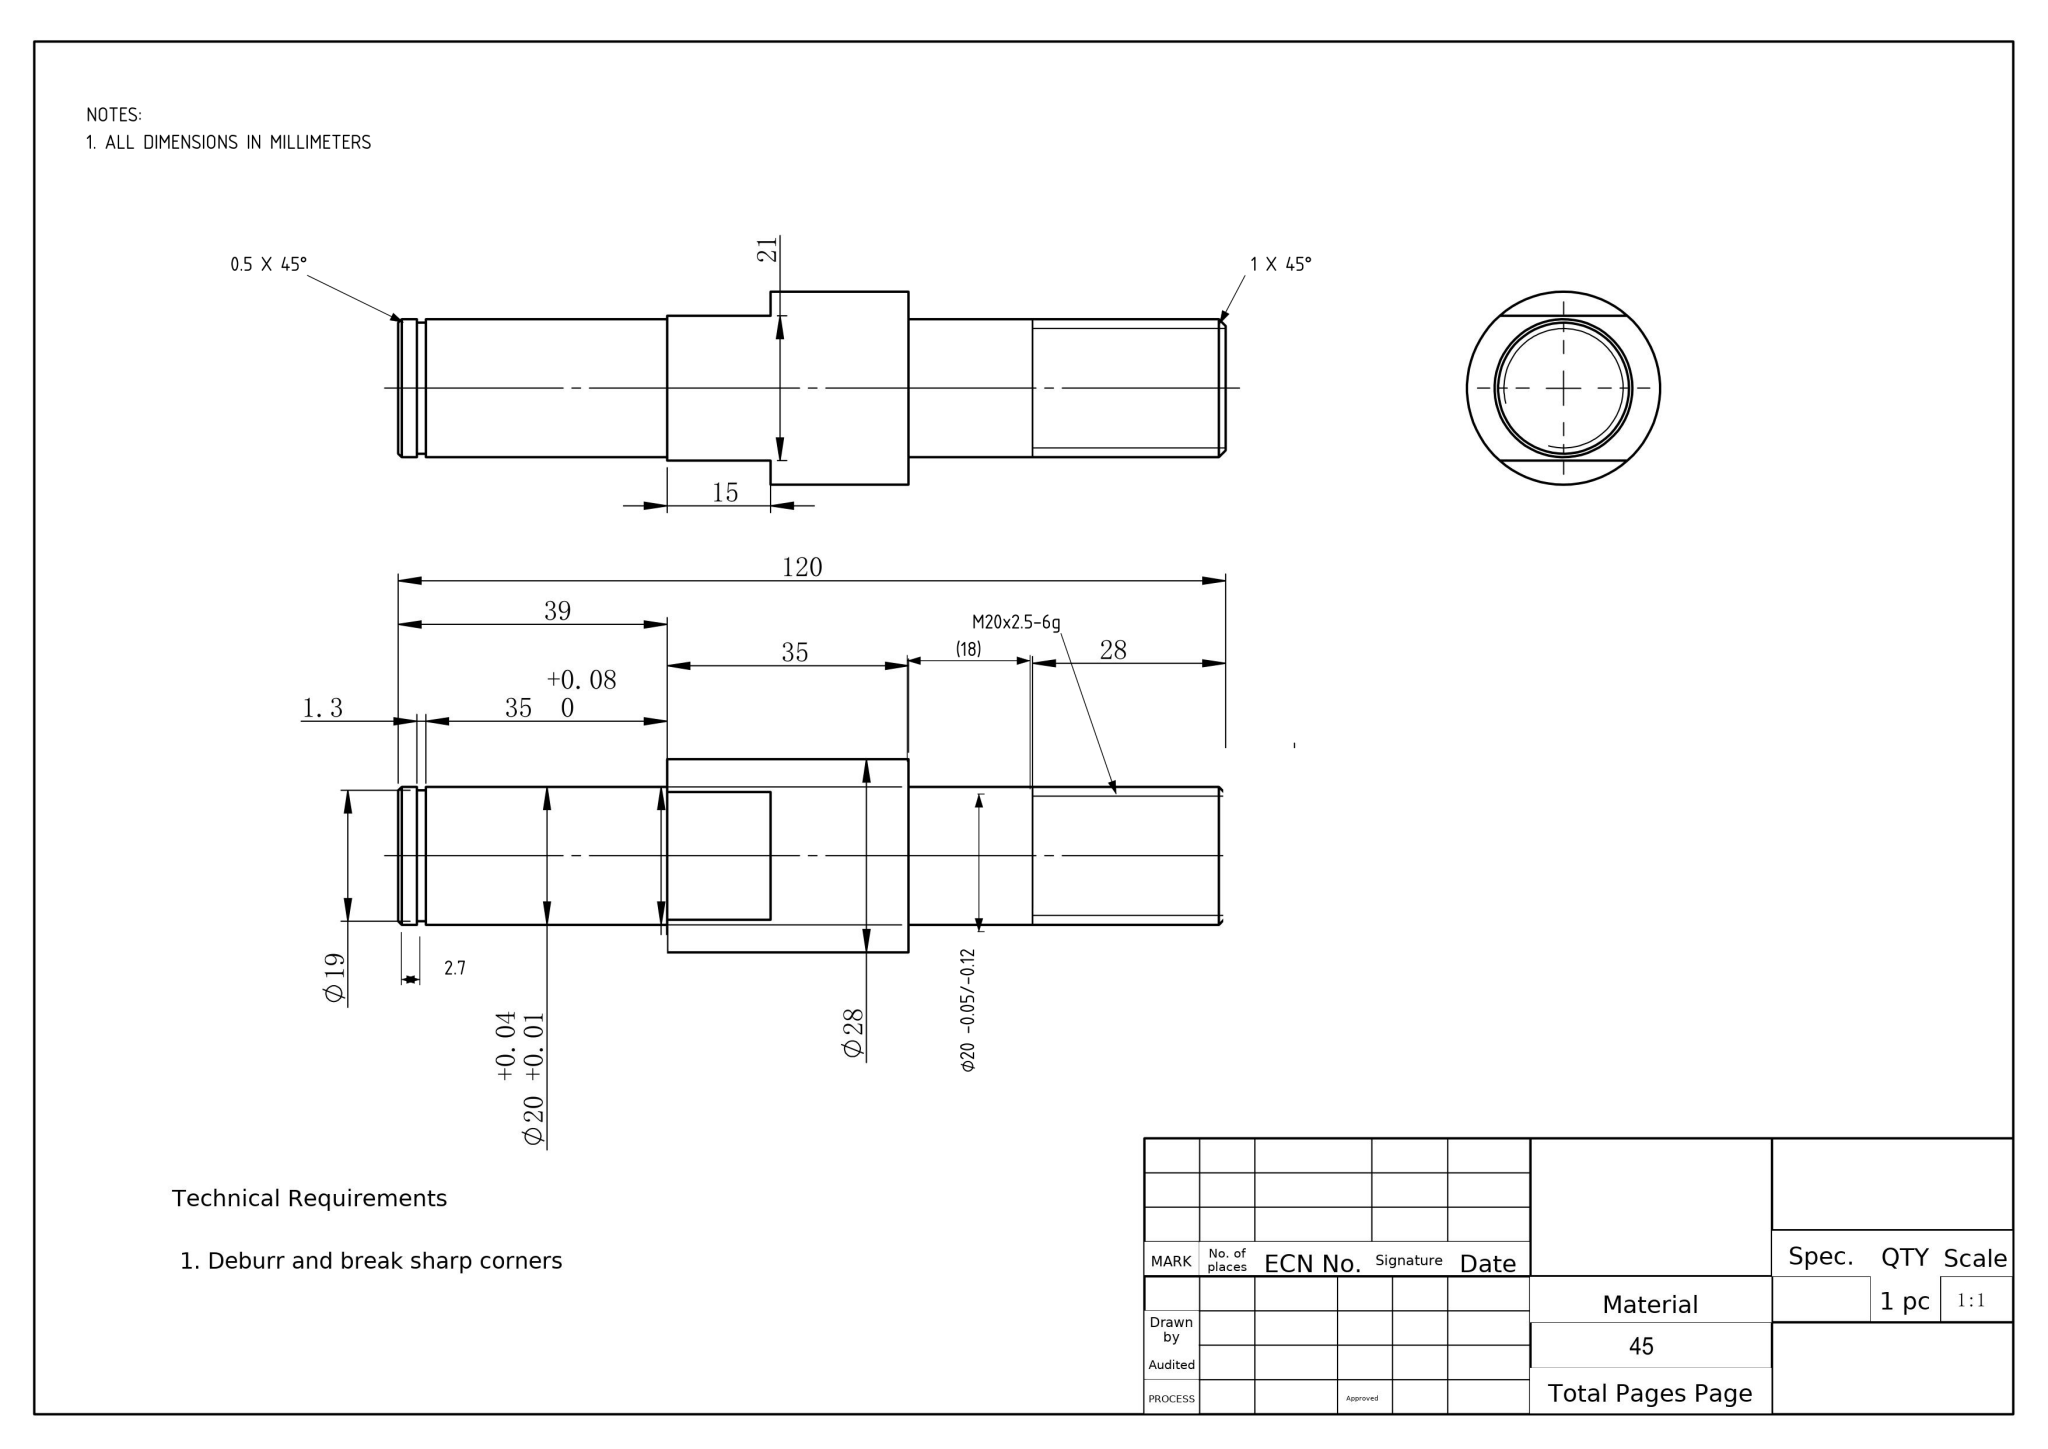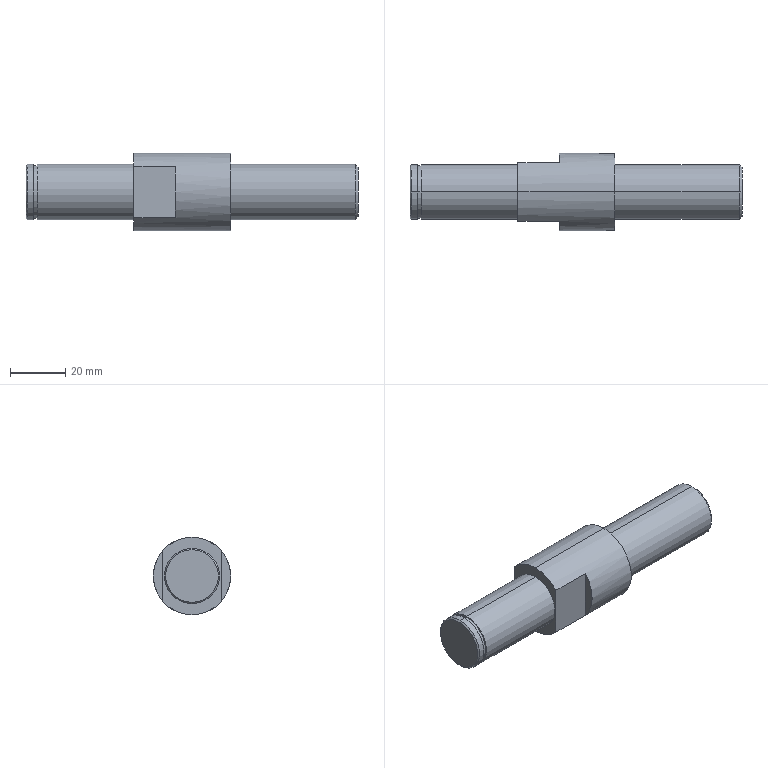Part | NX | mm | 1 solid | 24 faces | box 120 x 28 x 28 mm | volume 46844 mm3 | cylinder 10 | plane 10 | cone 4 | commonest cylinder face diameters 20 x6 19 x2 28 x2
STEP:
#1=COLOUR_RGB('',1.,0.502,0.502);
#2=FILL_AREA_STYLE_COLOUR('',#1);
#3=FILL_AREA_STYLE('',(#2));
#4=SURFACE_STYLE_FILL_AREA(#3);
#5=SURFACE_SIDE_STYLE('',(#4));
#6=SURFACE_STYLE_USAGE(.BOTH.,#5);
#7=PRESENTATION_STYLE_ASSIGNMENT((#6));
#8=CARTESIAN_POINT('',(120.,0.,9.));
#9=VERTEX_POINT('',#8);
#10=CARTESIAN_POINT('',(120.,0.,-9.));
#11=VERTEX_POINT('',#10);
#12=CARTESIAN_POINT('',(120.,0.,0.));
#13=DIRECTION('',(-1.,0.,0.));
#14=DIRECTION('',(0.,0.,1.));
#15=AXIS2_PLACEMENT_3D('',#12,#13,#14);
#16=CIRCLE('',#15,9.);
#17=EDGE_CURVE('',#9,#11,#16,.T.);
#18=ORIENTED_EDGE('',*,*,#17,.T.);
#19=CARTESIAN_POINT('',(119.,0.,-10.));
#20=VERTEX_POINT('',#19);
#21=CARTESIAN_POINT('',(120.,0.,-9.));
#22=DIRECTION('',(-0.7071,0.,-0.7071));
#23=VECTOR('',#22,1000.);
#24=LINE('',#21,#23);
#25=EDGE_CURVE('',#11,#20,#24,.T.);
#26=ORIENTED_EDGE('',*,*,#25,.T.);
#27=CARTESIAN_POINT('',(119.,0.,10.));
#28=VERTEX_POINT('',#27);
#29=CARTESIAN_POINT('',(119.,0.,0.));
#30=DIRECTION('',(-1.,0.,0.));
#31=DIRECTION('',(0.,0.,1.));
#32=AXIS2_PLACEMENT_3D('',#29,#30,#31);
#33=CIRCLE('',#32,10.);
#34=EDGE_CURVE('',#28,#20,#33,.T.);
#35=ORIENTED_EDGE('',*,*,#34,.F.);
#36=CARTESIAN_POINT('',(120.,0.,9.));
#37=DIRECTION('',(-0.7071,0.,0.7071));
#38=VECTOR('',#37,1000.);
#39=LINE('',#36,#38);
#40=EDGE_CURVE('',#9,#28,#39,.T.);
#41=ORIENTED_EDGE('',*,*,#40,.F.);
#42=EDGE_LOOP('',(#18,#26,#35,#41));
#43=FACE_OUTER_BOUND('',#42,.T.);
#44=CARTESIAN_POINT('',(120.,0.,0.));
#45=DIRECTION('',(-1.,0.,0.));
#46=DIRECTION('',(0.,0.,1.));
#47=AXIS2_PLACEMENT_3D('',#44,#45,#46);
#48=CONICAL_SURFACE('',#47,9.,0.7854);
#49=ADVANCED_FACE('',(#43),#48,.T.);
#50=ORIENTED_EDGE('',*,*,#34,.T.);
#51=CARTESIAN_POINT('',(74.,0.,-10.));
#52=VERTEX_POINT('',#51);
#53=CARTESIAN_POINT('',(0.,0.,-10.));
#54=DIRECTION('',(-1.,0.,0.));
#55=VECTOR('',#54,1000.);
#56=LINE('',#53,#55);
#57=EDGE_CURVE('',#20,#52,#56,.T.);
#58=ORIENTED_EDGE('',*,*,#57,.T.);
#59=CARTESIAN_POINT('',(74.,0.,10.));
#60=VERTEX_POINT('',#59);
#61=CARTESIAN_POINT('',(74.,0.,0.));
#62=DIRECTION('',(-1.,0.,0.));
#63=DIRECTION('',(0.,0.,1.));
#64=AXIS2_PLACEMENT_3D('',#61,#62,#63);
#65=CIRCLE('',#64,10.);
#66=EDGE_CURVE('',#60,#52,#65,.T.);
#67=ORIENTED_EDGE('',*,*,#66,.F.);
#68=CARTESIAN_POINT('',(0.,0.,10.));
#69=DIRECTION('',(-1.,0.,0.));
#70=VECTOR('',#69,1000.);
#71=LINE('',#68,#70);
#72=EDGE_CURVE('',#28,#60,#71,.T.);
#73=ORIENTED_EDGE('',*,*,#72,.F.);
#74=EDGE_LOOP('',(#50,#58,#67,#73));
#75=FACE_OUTER_BOUND('',#74,.T.);
#76=CARTESIAN_POINT('',(0.,0.,0.));
#77=DIRECTION('',(-1.,0.,0.));
#78=DIRECTION('',(0.,0.,1.));
#79=AXIS2_PLACEMENT_3D('',#76,#77,#78);
#80=CYLINDRICAL_SURFACE('',#79,10.);
#81=ADVANCED_FACE('',(#75),#80,.T.);
#82=CARTESIAN_POINT('',(39.,0.,10.));
#83=VERTEX_POINT('',#82);
#84=CARTESIAN_POINT('',(39.,0.,-10.));
#85=VERTEX_POINT('',#84);
#86=CARTESIAN_POINT('',(39.,0.,0.));
#87=DIRECTION('',(-1.,0.,0.));
#88=DIRECTION('',(0.,0.,1.));
#89=AXIS2_PLACEMENT_3D('',#86,#87,#88);
#90=CIRCLE('',#89,10.);
#91=EDGE_CURVE('',#83,#85,#90,.T.);
#92=ORIENTED_EDGE('',*,*,#91,.T.);
#93=CARTESIAN_POINT('',(4.,0.,-10.));
#94=VERTEX_POINT('',#93);
#95=CARTESIAN_POINT('',(0.,0.,-10.));
#96=DIRECTION('',(-1.,0.,0.));
#97=VECTOR('',#96,1000.);
#98=LINE('',#95,#97);
#99=EDGE_CURVE('',#85,#94,#98,.T.);
#100=ORIENTED_EDGE('',*,*,#99,.T.);
#101=CARTESIAN_POINT('',(4.,0.,10.));
#102=VERTEX_POINT('',#101);
#103=CARTESIAN_POINT('',(4.,0.,0.));
#104=DIRECTION('',(-1.,0.,0.));
#105=DIRECTION('',(0.,0.,1.));
#106=AXIS2_PLACEMENT_3D('',#103,#104,#105);
#107=CIRCLE('',#106,10.);
#108=EDGE_CURVE('',#102,#94,#107,.T.);
#109=ORIENTED_EDGE('',*,*,#108,.F.);
#110=CARTESIAN_POINT('',(0.,0.,10.));
#111=DIRECTION('',(-1.,0.,0.));
#112=VECTOR('',#111,1000.);
#113=LINE('',#110,#112);
#114=EDGE_CURVE('',#83,#102,#113,.T.);
#115=ORIENTED_EDGE('',*,*,#114,.F.);
#116=EDGE_LOOP('',(#92,#100,#109,#115));
#117=FACE_OUTER_BOUND('',#116,.T.);
#118=CARTESIAN_POINT('',(0.,0.,0.));
#119=DIRECTION('',(-1.,0.,0.));
#120=DIRECTION('',(0.,0.,1.));
#121=AXIS2_PLACEMENT_3D('',#118,#119,#120);
#122=CYLINDRICAL_SURFACE('',#121,10.);
#123=ADVANCED_FACE('',(#117),#122,.T.);
#124=CARTESIAN_POINT('',(4.,0.,9.5));
#125=VERTEX_POINT('',#124);
#126=CARTESIAN_POINT('',(4.,0.,-9.5));
#127=VERTEX_POINT('',#126);
#128=CARTESIAN_POINT('',(4.,0.,0.));
#129=DIRECTION('',(-1.,0.,0.));
#130=DIRECTION('',(0.,0.,1.));
#131=AXIS2_PLACEMENT_3D('',#128,#129,#130);
#132=CIRCLE('',#131,9.5);
#133=EDGE_CURVE('',#125,#127,#132,.T.);
#134=ORIENTED_EDGE('',*,*,#133,.T.);
#135=CARTESIAN_POINT('',(2.7,0.,-9.5));
#136=VERTEX_POINT('',#135);
#137=CARTESIAN_POINT('',(0.,0.,-9.5));
#138=DIRECTION('',(-1.,0.,0.));
#139=VECTOR('',#138,1000.);
#140=LINE('',#137,#139);
#141=EDGE_CURVE('',#127,#136,#140,.T.);
#142=ORIENTED_EDGE('',*,*,#141,.T.);
#143=CARTESIAN_POINT('',(2.7,0.,9.5));
#144=VERTEX_POINT('',#143);
#145=CARTESIAN_POINT('',(2.7,0.,0.));
#146=DIRECTION('',(-1.,0.,0.));
#147=DIRECTION('',(0.,0.,1.));
#148=AXIS2_PLACEMENT_3D('',#145,#146,#147);
#149=CIRCLE('',#148,9.5);
#150=EDGE_CURVE('',#144,#136,#149,.T.);
#151=ORIENTED_EDGE('',*,*,#150,.F.);
#152=CARTESIAN_POINT('',(0.,0.,9.5));
#153=DIRECTION('',(-1.,0.,0.));
#154=VECTOR('',#153,1000.);
#155=LINE('',#152,#154);
#156=EDGE_CURVE('',#125,#144,#155,.T.);
#157=ORIENTED_EDGE('',*,*,#156,.F.);
#158=EDGE_LOOP('',(#134,#142,#151,#157));
#159=FACE_OUTER_BOUND('',#158,.T.);
#160=CARTESIAN_POINT('',(0.,0.,0.));
#161=DIRECTION('',(-1.,0.,0.));
#162=DIRECTION('',(0.,0.,1.));
#163=AXIS2_PLACEMENT_3D('',#160,#161,#162);
#164=CYLINDRICAL_SURFACE('',#163,9.5);
#165=ADVANCED_FACE('',(#159),#164,.T.);
#166=CARTESIAN_POINT('',(2.7,0.,10.));
#167=VERTEX_POINT('',#166);
#168=CARTESIAN_POINT('',(2.7,0.,-10.));
#169=VERTEX_POINT('',#168);
#170=CARTESIAN_POINT('',(2.7,0.,0.));
#171=DIRECTION('',(-1.,0.,0.));
#172=DIRECTION('',(0.,0.,1.));
#173=AXIS2_PLACEMENT_3D('',#170,#171,#172);
#174=CIRCLE('',#173,10.);
#175=EDGE_CURVE('',#167,#169,#174,.T.);
#176=ORIENTED_EDGE('',*,*,#175,.T.);
#177=CARTESIAN_POINT('',(0.5,0.,-10.));
#178=VERTEX_POINT('',#177);
#179=CARTESIAN_POINT('',(0.,0.,-10.));
#180=DIRECTION('',(-1.,0.,0.));
#181=VECTOR('',#180,1000.);
#182=LINE('',#179,#181);
#183=EDGE_CURVE('',#169,#178,#182,.T.);
#184=ORIENTED_EDGE('',*,*,#183,.T.);
#185=CARTESIAN_POINT('',(0.5,0.,10.));
#186=VERTEX_POINT('',#185);
#187=CARTESIAN_POINT('',(0.5,0.,0.));
#188=DIRECTION('',(-1.,0.,0.));
#189=DIRECTION('',(0.,0.,1.));
#190=AXIS2_PLACEMENT_3D('',#187,#188,#189);
#191=CIRCLE('',#190,10.);
#192=EDGE_CURVE('',#186,#178,#191,.T.);
#193=ORIENTED_EDGE('',*,*,#192,.F.);
#194=CARTESIAN_POINT('',(0.,0.,10.));
#195=DIRECTION('',(-1.,0.,0.));
#196=VECTOR('',#195,1000.);
#197=LINE('',#194,#196);
#198=EDGE_CURVE('',#167,#186,#197,.T.);
#199=ORIENTED_EDGE('',*,*,#198,.F.);
#200=EDGE_LOOP('',(#176,#184,#193,#199));
#201=FACE_OUTER_BOUND('',#200,.T.);
#202=CARTESIAN_POINT('',(0.,0.,0.));
#203=DIRECTION('',(-1.,0.,0.));
#204=DIRECTION('',(0.,0.,1.));
#205=AXIS2_PLACEMENT_3D('',#202,#203,#204);
#206=CYLINDRICAL_SURFACE('',#205,10.);
#207=ADVANCED_FACE('',(#201),#206,.T.);
#208=CARTESIAN_POINT('',(0.,0.,9.5));
#209=VERTEX_POINT('',#208);
#210=CARTESIAN_POINT('',(0.,0.,-9.5));
#211=VERTEX_POINT('',#210);
#212=CARTESIAN_POINT('',(0.,0.,0.));
#213=DIRECTION('',(-1.,0.,0.));
#214=DIRECTION('',(0.,0.,1.));
#215=AXIS2_PLACEMENT_3D('',#212,#213,#214);
#216=CIRCLE('',#215,9.5);
#217=EDGE_CURVE('',#209,#211,#216,.T.);
#218=ORIENTED_EDGE('',*,*,#217,.F.);
#219=CARTESIAN_POINT('',(0.5,0.,10.));
#220=DIRECTION('',(0.7071,0.,0.7071));
#221=VECTOR('',#220,1000.);
#222=LINE('',#219,#221);
#223=EDGE_CURVE('',#209,#186,#222,.T.);
#224=ORIENTED_EDGE('',*,*,#223,.T.);
#225=ORIENTED_EDGE('',*,*,#192,.T.);
#226=CARTESIAN_POINT('',(0.5,0.,-10.));
#227=DIRECTION('',(0.7071,0.,-0.7071));
#228=VECTOR('',#227,1000.);
#229=LINE('',#226,#228);
#230=EDGE_CURVE('',#211,#178,#229,.T.);
#231=ORIENTED_EDGE('',*,*,#230,.F.);
#232=EDGE_LOOP('',(#218,#224,#225,#231));
#233=FACE_OUTER_BOUND('',#232,.T.);
#234=CARTESIAN_POINT('',(0.5,0.,0.));
#235=DIRECTION('',(1.,0.,0.));
#236=DIRECTION('',(0.,0.,-1.));
#237=AXIS2_PLACEMENT_3D('',#234,#235,#236);
#238=CONICAL_SURFACE('',#237,10.,0.7854);
#239=ADVANCED_FACE('',(#233),#238,.T.);
#240=CARTESIAN_POINT('',(74.,0.,14.));
#241=VERTEX_POINT('',#240);
#242=CARTESIAN_POINT('',(74.,0.,-14.));
#243=VERTEX_POINT('',#242);
#244=CARTESIAN_POINT('',(74.,0.,0.));
#245=DIRECTION('',(-1.,0.,0.));
#246=DIRECTION('',(0.,0.,1.));
#247=AXIS2_PLACEMENT_3D('',#244,#245,#246);
#248=CIRCLE('',#247,14.);
#249=EDGE_CURVE('',#241,#243,#248,.T.);
#250=ORIENTED_EDGE('',*,*,#249,.T.);
#251=CARTESIAN_POINT('',(39.,0.,-14.));
#252=VERTEX_POINT('',#251);
#253=CARTESIAN_POINT('',(0.,0.,-14.));
#254=DIRECTION('',(-1.,0.,0.));
#255=VECTOR('',#254,1000.);
#256=LINE('',#253,#255);
#257=EDGE_CURVE('',#243,#252,#256,.T.);
#258=ORIENTED_EDGE('',*,*,#257,.T.);
#259=CARTESIAN_POINT('',(39.,10.5,-9.26));
#260=VERTEX_POINT('',#259);
#261=CARTESIAN_POINT('',(39.,0.,0.));
#262=DIRECTION('',(-1.,0.,0.));
#263=DIRECTION('',(0.,0.,1.));
#264=AXIS2_PLACEMENT_3D('',#261,#262,#263);
#265=CIRCLE('',#264,14.);
#266=EDGE_CURVE('',#260,#252,#265,.T.);
#267=ORIENTED_EDGE('',*,*,#266,.F.);
#268=CARTESIAN_POINT('',(54.,10.5,-9.26));
#269=VERTEX_POINT('',#268);
#270=CARTESIAN_POINT('',(0.,10.5,-9.26));
#271=DIRECTION('',(-1.,0.,0.));
#272=VECTOR('',#271,1000.);
#273=LINE('',#270,#272);
#274=EDGE_CURVE('',#269,#260,#273,.T.);
#275=ORIENTED_EDGE('',*,*,#274,.F.);
#276=CARTESIAN_POINT('',(54.,10.5,9.26));
#277=VERTEX_POINT('',#276);
#278=CARTESIAN_POINT('',(54.,0.,0.));
#279=DIRECTION('',(-1.,0.,0.));
#280=DIRECTION('',(0.,0.,1.));
#281=AXIS2_PLACEMENT_3D('',#278,#279,#280);
#282=CIRCLE('',#281,14.);
#283=EDGE_CURVE('',#277,#269,#282,.T.);
#284=ORIENTED_EDGE('',*,*,#283,.F.);
#285=CARTESIAN_POINT('',(39.,10.5,9.26));
#286=VERTEX_POINT('',#285);
#287=CARTESIAN_POINT('',(0.,10.5,9.26));
#288=DIRECTION('',(1.,0.,0.));
#289=VECTOR('',#288,1000.);
#290=LINE('',#287,#289);
#291=EDGE_CURVE('',#286,#277,#290,.T.);
#292=ORIENTED_EDGE('',*,*,#291,.F.);
#293=CARTESIAN_POINT('',(39.,0.,14.));
#294=VERTEX_POINT('',#293);
#295=CARTESIAN_POINT('',(39.,0.,0.));
#296=DIRECTION('',(-1.,0.,0.));
#297=DIRECTION('',(0.,0.,1.));
#298=AXIS2_PLACEMENT_3D('',#295,#296,#297);
#299=CIRCLE('',#298,14.);
#300=EDGE_CURVE('',#294,#286,#299,.T.);
#301=ORIENTED_EDGE('',*,*,#300,.F.);
#302=CARTESIAN_POINT('',(0.,0.,14.));
#303=DIRECTION('',(-1.,0.,0.));
#304=VECTOR('',#303,1000.);
#305=LINE('',#302,#304);
#306=EDGE_CURVE('',#241,#294,#305,.T.);
#307=ORIENTED_EDGE('',*,*,#306,.F.);
#308=EDGE_LOOP('',(#250,#258,#267,#275,#284,#292,#301,#307));
#309=FACE_OUTER_BOUND('',#308,.T.);
#310=CARTESIAN_POINT('',(0.,0.,0.));
#311=DIRECTION('',(-1.,0.,0.));
#312=DIRECTION('',(0.,0.,1.));
#313=AXIS2_PLACEMENT_3D('',#310,#311,#312);
#314=CYLINDRICAL_SURFACE('',#313,14.);
#315=ADVANCED_FACE('',(#309),#314,.T.);
#316=ORIENTED_EDGE('',*,*,#91,.F.);
#317=CARTESIAN_POINT('',(39.,0.,0.));
#318=DIRECTION('',(-1.,0.,0.));
#319=DIRECTION('',(0.,0.,1.));
#320=AXIS2_PLACEMENT_3D('',#317,#318,#319);
#321=CIRCLE('',#320,10.);
#322=EDGE_CURVE('',#85,#83,#321,.T.);
#323=ORIENTED_EDGE('',*,*,#322,.F.);
#324=EDGE_LOOP('',(#316,#323));
#325=FACE_BOUND('',#324,.T.);
#326=CARTESIAN_POINT('',(39.,-10.5,-9.26));
#327=VERTEX_POINT('',#326);
#328=CARTESIAN_POINT('',(39.,-10.5,9.26));
#329=VERTEX_POINT('',#328);
#330=CARTESIAN_POINT('',(39.,-10.5,-15.599));
#331=DIRECTION('',(0.,0.,1.));
#332=VECTOR('',#331,1000.);
#333=LINE('',#330,#332);
#334=EDGE_CURVE('',#327,#329,#333,.T.);
#335=ORIENTED_EDGE('',*,*,#334,.T.);
#336=CARTESIAN_POINT('',(39.,0.,0.));
#337=DIRECTION('',(-1.,0.,0.));
#338=DIRECTION('',(0.,0.,1.));
#339=AXIS2_PLACEMENT_3D('',#336,#337,#338);
#340=CIRCLE('',#339,14.);
#341=EDGE_CURVE('',#329,#294,#340,.T.);
#342=ORIENTED_EDGE('',*,*,#341,.T.);
#343=ORIENTED_EDGE('',*,*,#300,.T.);
#344=CARTESIAN_POINT('',(39.,10.5,-15.599));
#345=DIRECTION('',(0.,0.,-1.));
#346=VECTOR('',#345,1000.);
#347=LINE('',#344,#346);
#348=EDGE_CURVE('',#286,#260,#347,.T.);
#349=ORIENTED_EDGE('',*,*,#348,.T.);
#350=ORIENTED_EDGE('',*,*,#266,.T.);
#351=CARTESIAN_POINT('',(39.,0.,0.));
#352=DIRECTION('',(-1.,0.,0.));
#353=DIRECTION('',(0.,0.,1.));
#354=AXIS2_PLACEMENT_3D('',#351,#352,#353);
#355=CIRCLE('',#354,14.);
#356=EDGE_CURVE('',#252,#327,#355,.T.);
#357=ORIENTED_EDGE('',*,*,#356,.T.);
#358=EDGE_LOOP('',(#335,#342,#343,#349,#350,#357));
#359=FACE_OUTER_BOUND('',#358,.T.);
#360=CARTESIAN_POINT('',(39.,10.,0.));
#361=DIRECTION('',(1.,0.,0.));
#362=DIRECTION('',(0.,0.,-1.));
#363=AXIS2_PLACEMENT_3D('',#360,#361,#362);
#364=PLANE('',#363);
#365=ADVANCED_FACE('',(#325,#359),#364,.F.);
#366=ORIENTED_EDGE('',*,*,#257,.F.);
#367=CARTESIAN_POINT('',(74.,0.,0.));
#368=DIRECTION('',(-1.,0.,0.));
#369=DIRECTION('',(0.,0.,1.));
#370=AXIS2_PLACEMENT_3D('',#367,#368,#369);
#371=CIRCLE('',#370,14.);
#372=EDGE_CURVE('',#243,#241,#371,.T.);
#373=ORIENTED_EDGE('',*,*,#372,.T.);
#374=ORIENTED_EDGE('',*,*,#306,.T.);
#375=ORIENTED_EDGE('',*,*,#341,.F.);
#376=CARTESIAN_POINT('',(54.,-10.5,9.26));
#377=VERTEX_POINT('',#376);
#378=CARTESIAN_POINT('',(0.,-10.5,9.26));
#379=DIRECTION('',(-1.,0.,0.));
#380=VECTOR('',#379,1000.);
#381=LINE('',#378,#380);
#382=EDGE_CURVE('',#377,#329,#381,.T.);
#383=ORIENTED_EDGE('',*,*,#382,.F.);
#384=CARTESIAN_POINT('',(54.,-10.5,-9.26));
#385=VERTEX_POINT('',#384);
#386=CARTESIAN_POINT('',(54.,0.,0.));
#387=DIRECTION('',(-1.,0.,0.));
#388=DIRECTION('',(0.,0.,1.));
#389=AXIS2_PLACEMENT_3D('',#386,#387,#388);
#390=CIRCLE('',#389,14.);
#391=EDGE_CURVE('',#385,#377,#390,.T.);
#392=ORIENTED_EDGE('',*,*,#391,.F.);
#393=CARTESIAN_POINT('',(0.,-10.5,-9.26));
#394=DIRECTION('',(1.,0.,0.));
#395=VECTOR('',#394,1000.);
#396=LINE('',#393,#395);
#397=EDGE_CURVE('',#327,#385,#396,.T.);
#398=ORIENTED_EDGE('',*,*,#397,.F.);
#399=ORIENTED_EDGE('',*,*,#356,.F.);
#400=EDGE_LOOP('',(#366,#373,#374,#375,#383,#392,#398,#399));
#401=FACE_OUTER_BOUND('',#400,.T.);
#402=CARTESIAN_POINT('',(0.,0.,0.));
#403=DIRECTION('',(-1.,0.,0.));
#404=DIRECTION('',(0.,0.,1.));
#405=AXIS2_PLACEMENT_3D('',#402,#403,#404);
#406=CYLINDRICAL_SURFACE('',#405,14.);
#407=ADVANCED_FACE('',(#401),#406,.T.);
#408=CARTESIAN_POINT('',(0.,0.,0.));
#409=DIRECTION('',(-1.,0.,0.));
#410=DIRECTION('',(0.,0.,1.));
#411=AXIS2_PLACEMENT_3D('',#408,#409,#410);
#412=CIRCLE('',#411,9.5);
#413=EDGE_CURVE('',#211,#209,#412,.T.);
#414=ORIENTED_EDGE('',*,*,#413,.T.);
#415=ORIENTED_EDGE('',*,*,#217,.T.);
#416=EDGE_LOOP('',(#414,#415));
#417=FACE_OUTER_BOUND('',#416,.T.);
#418=CARTESIAN_POINT('',(0.,0.,0.));
#419=DIRECTION('',(1.,0.,0.));
#420=DIRECTION('',(0.,0.,-1.));
#421=AXIS2_PLACEMENT_3D('',#418,#419,#420);
#422=PLANE('',#421);
#423=ADVANCED_FACE('',(#417),#422,.F.);
#424=ORIENTED_EDGE('',*,*,#223,.F.);
#425=ORIENTED_EDGE('',*,*,#413,.F.);
#426=ORIENTED_EDGE('',*,*,#230,.T.);
#427=CARTESIAN_POINT('',(0.5,0.,0.));
#428=DIRECTION('',(-1.,0.,0.));
#429=DIRECTION('',(0.,0.,1.));
#430=AXIS2_PLACEMENT_3D('',#427,#428,#429);
#431=CIRCLE('',#430,10.);
#432=EDGE_CURVE('',#178,#186,#431,.T.);
#433=ORIENTED_EDGE('',*,*,#432,.T.);
#434=EDGE_LOOP('',(#424,#425,#426,#433));
#435=FACE_OUTER_BOUND('',#434,.T.);
#436=CARTESIAN_POINT('',(0.5,0.,0.));
#437=DIRECTION('',(1.,0.,0.));
#438=DIRECTION('',(0.,0.,-1.));
#439=AXIS2_PLACEMENT_3D('',#436,#437,#438);
#440=CONICAL_SURFACE('',#439,10.,0.7854);
#441=ADVANCED_FACE('',(#435),#440,.T.);
#442=ORIENTED_EDGE('',*,*,#183,.F.);
#443=CARTESIAN_POINT('',(2.7,0.,0.));
#444=DIRECTION('',(-1.,0.,0.));
#445=DIRECTION('',(0.,0.,1.));
#446=AXIS2_PLACEMENT_3D('',#443,#444,#445);
#447=CIRCLE('',#446,10.);
#448=EDGE_CURVE('',#169,#167,#447,.T.);
#449=ORIENTED_EDGE('',*,*,#448,.T.);
#450=ORIENTED_EDGE('',*,*,#198,.T.);
#451=ORIENTED_EDGE('',*,*,#432,.F.);
#452=EDGE_LOOP('',(#442,#449,#450,#451));
#453=FACE_OUTER_BOUND('',#452,.T.);
#454=CARTESIAN_POINT('',(0.,0.,0.));
#455=DIRECTION('',(-1.,0.,0.));
#456=DIRECTION('',(0.,0.,1.));
#457=AXIS2_PLACEMENT_3D('',#454,#455,#456);
#458=CYLINDRICAL_SURFACE('',#457,10.);
#459=ADVANCED_FACE('',(#453),#458,.T.);
#460=ORIENTED_EDGE('',*,*,#175,.F.);
#461=ORIENTED_EDGE('',*,*,#448,.F.);
#462=EDGE_LOOP('',(#460,#461));
#463=FACE_OUTER_BOUND('',#462,.T.);
#464=ORIENTED_EDGE('',*,*,#150,.T.);
#465=CARTESIAN_POINT('',(2.7,0.,0.));
#466=DIRECTION('',(-1.,0.,0.));
#467=DIRECTION('',(0.,0.,1.));
#468=AXIS2_PLACEMENT_3D('',#465,#466,#467);
#469=CIRCLE('',#468,9.5);
#470=EDGE_CURVE('',#136,#144,#469,.T.);
#471=ORIENTED_EDGE('',*,*,#470,.T.);
#472=EDGE_LOOP('',(#464,#471));
#473=FACE_BOUND('',#472,.T.);
#474=CARTESIAN_POINT('',(2.7,10.,0.));
#475=DIRECTION('',(-1.,0.,0.));
#476=DIRECTION('',(0.,0.,1.));
#477=AXIS2_PLACEMENT_3D('',#474,#475,#476);
#478=PLANE('',#477);
#479=ADVANCED_FACE('',(#463,#473),#478,.F.);
#480=ORIENTED_EDGE('',*,*,#141,.F.);
#481=CARTESIAN_POINT('',(4.,0.,0.));
#482=DIRECTION('',(-1.,0.,0.));
#483=DIRECTION('',(0.,0.,1.));
#484=AXIS2_PLACEMENT_3D('',#481,#482,#483);
#485=CIRCLE('',#484,9.5);
#486=EDGE_CURVE('',#127,#125,#485,.T.);
#487=ORIENTED_EDGE('',*,*,#486,.T.);
#488=ORIENTED_EDGE('',*,*,#156,.T.);
#489=ORIENTED_EDGE('',*,*,#470,.F.);
#490=EDGE_LOOP('',(#480,#487,#488,#489));
#491=FACE_OUTER_BOUND('',#490,.T.);
#492=CARTESIAN_POINT('',(0.,0.,0.));
#493=DIRECTION('',(-1.,0.,0.));
#494=DIRECTION('',(0.,0.,1.));
#495=AXIS2_PLACEMENT_3D('',#492,#493,#494);
#496=CYLINDRICAL_SURFACE('',#495,9.5);
#497=ADVANCED_FACE('',(#491),#496,.T.);
#498=ORIENTED_EDGE('',*,*,#133,.F.);
#499=ORIENTED_EDGE('',*,*,#486,.F.);
#500=EDGE_LOOP('',(#498,#499));
#501=FACE_BOUND('',#500,.T.);
#502=ORIENTED_EDGE('',*,*,#108,.T.);
#503=CARTESIAN_POINT('',(4.,0.,0.));
#504=DIRECTION('',(-1.,0.,0.));
#505=DIRECTION('',(0.,0.,1.));
#506=AXIS2_PLACEMENT_3D('',#503,#504,#505);
#507=CIRCLE('',#506,10.);
#508=EDGE_CURVE('',#94,#102,#507,.T.);
#509=ORIENTED_EDGE('',*,*,#508,.T.);
#510=EDGE_LOOP('',(#502,#509));
#511=FACE_OUTER_BOUND('',#510,.T.);
#512=CARTESIAN_POINT('',(4.,9.5,0.));
#513=DIRECTION('',(1.,0.,0.));
#514=DIRECTION('',(0.,0.,-1.));
#515=AXIS2_PLACEMENT_3D('',#512,#513,#514);
#516=PLANE('',#515);
#517=ADVANCED_FACE('',(#501,#511),#516,.F.);
#518=ORIENTED_EDGE('',*,*,#99,.F.);
#519=ORIENTED_EDGE('',*,*,#322,.T.);
#520=ORIENTED_EDGE('',*,*,#114,.T.);
#521=ORIENTED_EDGE('',*,*,#508,.F.);
#522=EDGE_LOOP('',(#518,#519,#520,#521));
#523=FACE_OUTER_BOUND('',#522,.T.);
#524=CARTESIAN_POINT('',(0.,0.,0.));
#525=DIRECTION('',(-1.,0.,0.));
#526=DIRECTION('',(0.,0.,1.));
#527=AXIS2_PLACEMENT_3D('',#524,#525,#526);
#528=CYLINDRICAL_SURFACE('',#527,10.);
#529=ADVANCED_FACE('',(#523),#528,.T.);
#530=ORIENTED_EDGE('',*,*,#249,.F.);
#531=ORIENTED_EDGE('',*,*,#372,.F.);
#532=EDGE_LOOP('',(#530,#531));
#533=FACE_OUTER_BOUND('',#532,.T.);
#534=ORIENTED_EDGE('',*,*,#66,.T.);
#535=CARTESIAN_POINT('',(74.,0.,0.));
#536=DIRECTION('',(-1.,0.,0.));
#537=DIRECTION('',(0.,0.,1.));
#538=AXIS2_PLACEMENT_3D('',#535,#536,#537);
#539=CIRCLE('',#538,10.);
#540=EDGE_CURVE('',#52,#60,#539,.T.);
#541=ORIENTED_EDGE('',*,*,#540,.T.);
#542=EDGE_LOOP('',(#534,#541));
#543=FACE_BOUND('',#542,.T.);
#544=CARTESIAN_POINT('',(74.,14.,0.));
#545=DIRECTION('',(-1.,0.,0.));
#546=DIRECTION('',(0.,0.,1.));
#547=AXIS2_PLACEMENT_3D('',#544,#545,#546);
#548=PLANE('',#547);
#549=ADVANCED_FACE('',(#533,#543),#548,.F.);
#550=ORIENTED_EDGE('',*,*,#57,.F.);
#551=CARTESIAN_POINT('',(119.,0.,0.));
#552=DIRECTION('',(-1.,0.,0.));
#553=DIRECTION('',(0.,0.,1.));
#554=AXIS2_PLACEMENT_3D('',#551,#552,#553);
#555=CIRCLE('',#554,10.);
#556=EDGE_CURVE('',#20,#28,#555,.T.);
#557=ORIENTED_EDGE('',*,*,#556,.T.);
#558=ORIENTED_EDGE('',*,*,#72,.T.);
#559=ORIENTED_EDGE('',*,*,#540,.F.);
#560=EDGE_LOOP('',(#550,#557,#558,#559));
#561=FACE_OUTER_BOUND('',#560,.T.);
#562=CARTESIAN_POINT('',(0.,0.,0.));
#563=DIRECTION('',(-1.,0.,0.));
#564=DIRECTION('',(0.,0.,1.));
#565=AXIS2_PLACEMENT_3D('',#562,#563,#564);
#566=CYLINDRICAL_SURFACE('',#565,10.);
#567=ADVANCED_FACE('',(#561),#566,.T.);
#568=ORIENTED_EDGE('',*,*,#25,.F.);
#569=CARTESIAN_POINT('',(120.,0.,0.));
#570=DIRECTION('',(-1.,0.,0.));
#571=DIRECTION('',(0.,0.,1.));
#572=AXIS2_PLACEMENT_3D('',#569,#570,#571);
#573=CIRCLE('',#572,9.);
#574=EDGE_CURVE('',#11,#9,#573,.T.);
#575=ORIENTED_EDGE('',*,*,#574,.T.);
#576=ORIENTED_EDGE('',*,*,#40,.T.);
#577=ORIENTED_EDGE('',*,*,#556,.F.);
#578=EDGE_LOOP('',(#568,#575,#576,#577));
#579=FACE_OUTER_BOUND('',#578,.T.);
#580=CARTESIAN_POINT('',(120.,0.,0.));
#581=DIRECTION('',(-1.,0.,0.));
#582=DIRECTION('',(0.,0.,1.));
#583=AXIS2_PLACEMENT_3D('',#580,#581,#582);
#584=CONICAL_SURFACE('',#583,9.,0.7854);
#585=ADVANCED_FACE('',(#579),#584,.T.);
#586=ORIENTED_EDGE('',*,*,#17,.F.);
#587=ORIENTED_EDGE('',*,*,#574,.F.);
#588=EDGE_LOOP('',(#586,#587));
#589=FACE_OUTER_BOUND('',#588,.T.);
#590=CARTESIAN_POINT('',(120.,9.,0.));
#591=DIRECTION('',(-1.,0.,0.));
#592=DIRECTION('',(0.,0.,1.));
#593=AXIS2_PLACEMENT_3D('',#590,#591,#592);
#594=PLANE('',#593);
#595=ADVANCED_FACE('',(#589),#594,.F.);
#596=ORIENTED_EDGE('',*,*,#274,.T.);
#597=ORIENTED_EDGE('',*,*,#348,.F.);
#598=ORIENTED_EDGE('',*,*,#291,.T.);
#599=CARTESIAN_POINT('',(54.,10.5,-15.599));
#600=DIRECTION('',(0.,0.,-1.));
#601=VECTOR('',#600,1000.);
#602=LINE('',#599,#601);
#603=EDGE_CURVE('',#277,#269,#602,.T.);
#604=ORIENTED_EDGE('',*,*,#603,.T.);
#605=EDGE_LOOP('',(#596,#597,#598,#604));
#606=FACE_OUTER_BOUND('',#605,.T.);
#607=CARTESIAN_POINT('',(54.,10.5,-15.599));
#608=DIRECTION('',(0.,1.,0.));
#609=DIRECTION('',(0.,0.,1.));
#610=AXIS2_PLACEMENT_3D('',#607,#608,#609);
#611=PLANE('',#610);
#612=ADVANCED_FACE('',(#606),#611,.T.);
#613=ORIENTED_EDGE('',*,*,#283,.T.);
#614=ORIENTED_EDGE('',*,*,#603,.F.);
#615=EDGE_LOOP('',(#613,#614));
#616=FACE_OUTER_BOUND('',#615,.T.);
#617=CARTESIAN_POINT('',(54.,0.,0.));
#618=DIRECTION('',(-1.,0.,0.));
#619=DIRECTION('',(0.,0.,1.));
#620=AXIS2_PLACEMENT_3D('',#617,#618,#619);
#621=PLANE('',#620);
#622=ADVANCED_FACE('',(#616),#621,.T.);
#623=ORIENTED_EDGE('',*,*,#391,.T.);
#624=CARTESIAN_POINT('',(54.,-10.5,-15.599));
#625=DIRECTION('',(0.,0.,1.));
#626=VECTOR('',#625,1000.);
#627=LINE('',#624,#626);
#628=EDGE_CURVE('',#385,#377,#627,.T.);
#629=ORIENTED_EDGE('',*,*,#628,.F.);
#630=EDGE_LOOP('',(#623,#629));
#631=FACE_OUTER_BOUND('',#630,.T.);
#632=CARTESIAN_POINT('',(54.,0.,0.));
#633=DIRECTION('',(-1.,0.,0.));
#634=DIRECTION('',(0.,0.,1.));
#635=AXIS2_PLACEMENT_3D('',#632,#633,#634);
#636=PLANE('',#635);
#637=ADVANCED_FACE('',(#631),#636,.T.);
#638=ORIENTED_EDGE('',*,*,#382,.T.);
#639=ORIENTED_EDGE('',*,*,#334,.F.);
#640=ORIENTED_EDGE('',*,*,#397,.T.);
#641=ORIENTED_EDGE('',*,*,#628,.T.);
#642=EDGE_LOOP('',(#638,#639,#640,#641));
#643=FACE_OUTER_BOUND('',#642,.T.);
#644=CARTESIAN_POINT('',(54.,-10.5,-15.599));
#645=DIRECTION('',(0.,-1.,0.));
#646=DIRECTION('',(0.,0.,-1.));
#647=AXIS2_PLACEMENT_3D('',#644,#645,#646);
#648=PLANE('',#647);
#649=ADVANCED_FACE('',(#643),#648,.T.);
#650=CLOSED_SHELL('',(#49,#81,#123,#165,#207,#239,#315,#365,#407,#423,#441,#459,#479,#497,#517,#529,#549,#567,#585,#595,#612,#622,#637,#649));
#651=MANIFOLD_SOLID_BREP('',#650);
#652=CARTESIAN_POINT('',(0.,0.,0.));
#653=DIRECTION('',(0.,0.,1.));
#654=DIRECTION('',(1.,0.,0.));
#655=AXIS2_PLACEMENT_3D('',#652,#653,#654);
#656=(LENGTH_UNIT()NAMED_UNIT(*)SI_UNIT(.MILLI.,.METRE.));
#657=UNCERTAINTY_MEASURE_WITH_UNIT(LENGTH_MEASURE(0.00001),#656,'','');
#658=(NAMED_UNIT(*)PLANE_ANGLE_UNIT()SI_UNIT($,.RADIAN.));
#659=(NAMED_UNIT(*)SI_UNIT($,.STERADIAN.)SOLID_ANGLE_UNIT());
#660=(GEOMETRIC_REPRESENTATION_CONTEXT(3)GLOBAL_UNCERTAINTY_ASSIGNED_CONTEXT((#657))GLOBAL_UNIT_ASSIGNED_CONTEXT((#656,#658,#659))REPRESENTATION_CONTEXT('',''));
#661=ADVANCED_BREP_SHAPE_REPRESENTATION('',(#651,#655),#660);
#662=STYLED_ITEM('',(#7),#661);
#663=(LENGTH_UNIT()NAMED_UNIT(*)SI_UNIT(.MILLI.,.METRE.));
#664=UNCERTAINTY_MEASURE_WITH_UNIT(LENGTH_MEASURE(0.00001),#663,'','');
#665=(NAMED_UNIT(*)PLANE_ANGLE_UNIT()SI_UNIT($,.RADIAN.));
#666=(NAMED_UNIT(*)SI_UNIT($,.STERADIAN.)SOLID_ANGLE_UNIT());
#667=(GEOMETRIC_REPRESENTATION_CONTEXT(3)GLOBAL_UNCERTAINTY_ASSIGNED_CONTEXT((#664))GLOBAL_UNIT_ASSIGNED_CONTEXT((#663,#665,#666))REPRESENTATION_CONTEXT('',''));
#668=MECHANICAL_DESIGN_GEOMETRIC_PRESENTATION_REPRESENTATION('',(#662),#667);
#669=PRESENTATION_LAYER_ASSIGNMENT('','',(#662));
#670=COLOUR_RGB('',1.,0.502,0.502);
#671=FILL_AREA_STYLE_COLOUR('',#670);
#672=FILL_AREA_STYLE('',(#671));
#673=SURFACE_STYLE_FILL_AREA(#672);
#674=SURFACE_SIDE_STYLE('',(#673));
#675=SURFACE_STYLE_USAGE(.BOTH.,#674);
#676=PRESENTATION_STYLE_ASSIGNMENT((#675));
#677=STYLED_ITEM('',(#676),#651);
#678=(LENGTH_UNIT()NAMED_UNIT(*)SI_UNIT(.MILLI.,.METRE.));
#679=UNCERTAINTY_MEASURE_WITH_UNIT(LENGTH_MEASURE(0.00001),#678,'','');
#680=(NAMED_UNIT(*)PLANE_ANGLE_UNIT()SI_UNIT($,.RADIAN.));
#681=(NAMED_UNIT(*)SI_UNIT($,.STERADIAN.)SOLID_ANGLE_UNIT());
#682=(GEOMETRIC_REPRESENTATION_CONTEXT(3)GLOBAL_UNCERTAINTY_ASSIGNED_CONTEXT((#679))GLOBAL_UNIT_ASSIGNED_CONTEXT((#678,#680,#681))REPRESENTATION_CONTEXT('',''));
#683=MECHANICAL_DESIGN_GEOMETRIC_PRESENTATION_REPRESENTATION('',(#677),#682);
#684=PRESENTATION_LAYER_ASSIGNMENT('','',(#677));
#685=COLOUR_RGB('',1.,0.502,0.502);
#686=FILL_AREA_STYLE_COLOUR('',#685);
#687=FILL_AREA_STYLE('',(#686));
#688=SURFACE_STYLE_FILL_AREA(#687);
#689=SURFACE_SIDE_STYLE('',(#688));
#690=SURFACE_STYLE_USAGE(.BOTH.,#689);
#691=PRESENTATION_STYLE_ASSIGNMENT((#690));
#692=STYLED_ITEM('',(#691),#81);
#693=(LENGTH_UNIT()NAMED_UNIT(*)SI_UNIT(.MILLI.,.METRE.));
#694=UNCERTAINTY_MEASURE_WITH_UNIT(LENGTH_MEASURE(0.00001),#693,'','');
#695=(NAMED_UNIT(*)PLANE_ANGLE_UNIT()SI_UNIT($,.RADIAN.));
#696=(NAMED_UNIT(*)SI_UNIT($,.STERADIAN.)SOLID_ANGLE_UNIT());
#697=(GEOMETRIC_REPRESENTATION_CONTEXT(3)GLOBAL_UNCERTAINTY_ASSIGNED_CONTEXT((#694))GLOBAL_UNIT_ASSIGNED_CONTEXT((#693,#695,#696))REPRESENTATION_CONTEXT('',''));
#698=MECHANICAL_DESIGN_GEOMETRIC_PRESENTATION_REPRESENTATION('',(#692),#697);
#699=PRESENTATION_LAYER_ASSIGNMENT('','',(#692));
#700=COLOUR_RGB('',1.,0.502,0.502);
#701=FILL_AREA_STYLE_COLOUR('',#700);
#702=FILL_AREA_STYLE('',(#701));
#703=SURFACE_STYLE_FILL_AREA(#702);
#704=SURFACE_SIDE_STYLE('',(#703));
#705=SURFACE_STYLE_USAGE(.BOTH.,#704);
#706=PRESENTATION_STYLE_ASSIGNMENT((#705));
#707=STYLED_ITEM('',(#706),#567);
#708=(LENGTH_UNIT()NAMED_UNIT(*)SI_UNIT(.MILLI.,.METRE.));
#709=UNCERTAINTY_MEASURE_WITH_UNIT(LENGTH_MEASURE(0.00001),#708,'','');
#710=(NAMED_UNIT(*)PLANE_ANGLE_UNIT()SI_UNIT($,.RADIAN.));
#711=(NAMED_UNIT(*)SI_UNIT($,.STERADIAN.)SOLID_ANGLE_UNIT());
#712=(GEOMETRIC_REPRESENTATION_CONTEXT(3)GLOBAL_UNCERTAINTY_ASSIGNED_CONTEXT((#709))GLOBAL_UNIT_ASSIGNED_CONTEXT((#708,#710,#711))REPRESENTATION_CONTEXT('',''));
#713=MECHANICAL_DESIGN_GEOMETRIC_PRESENTATION_REPRESENTATION('',(#707),#712);
#714=PRESENTATION_LAYER_ASSIGNMENT('','',(#707));